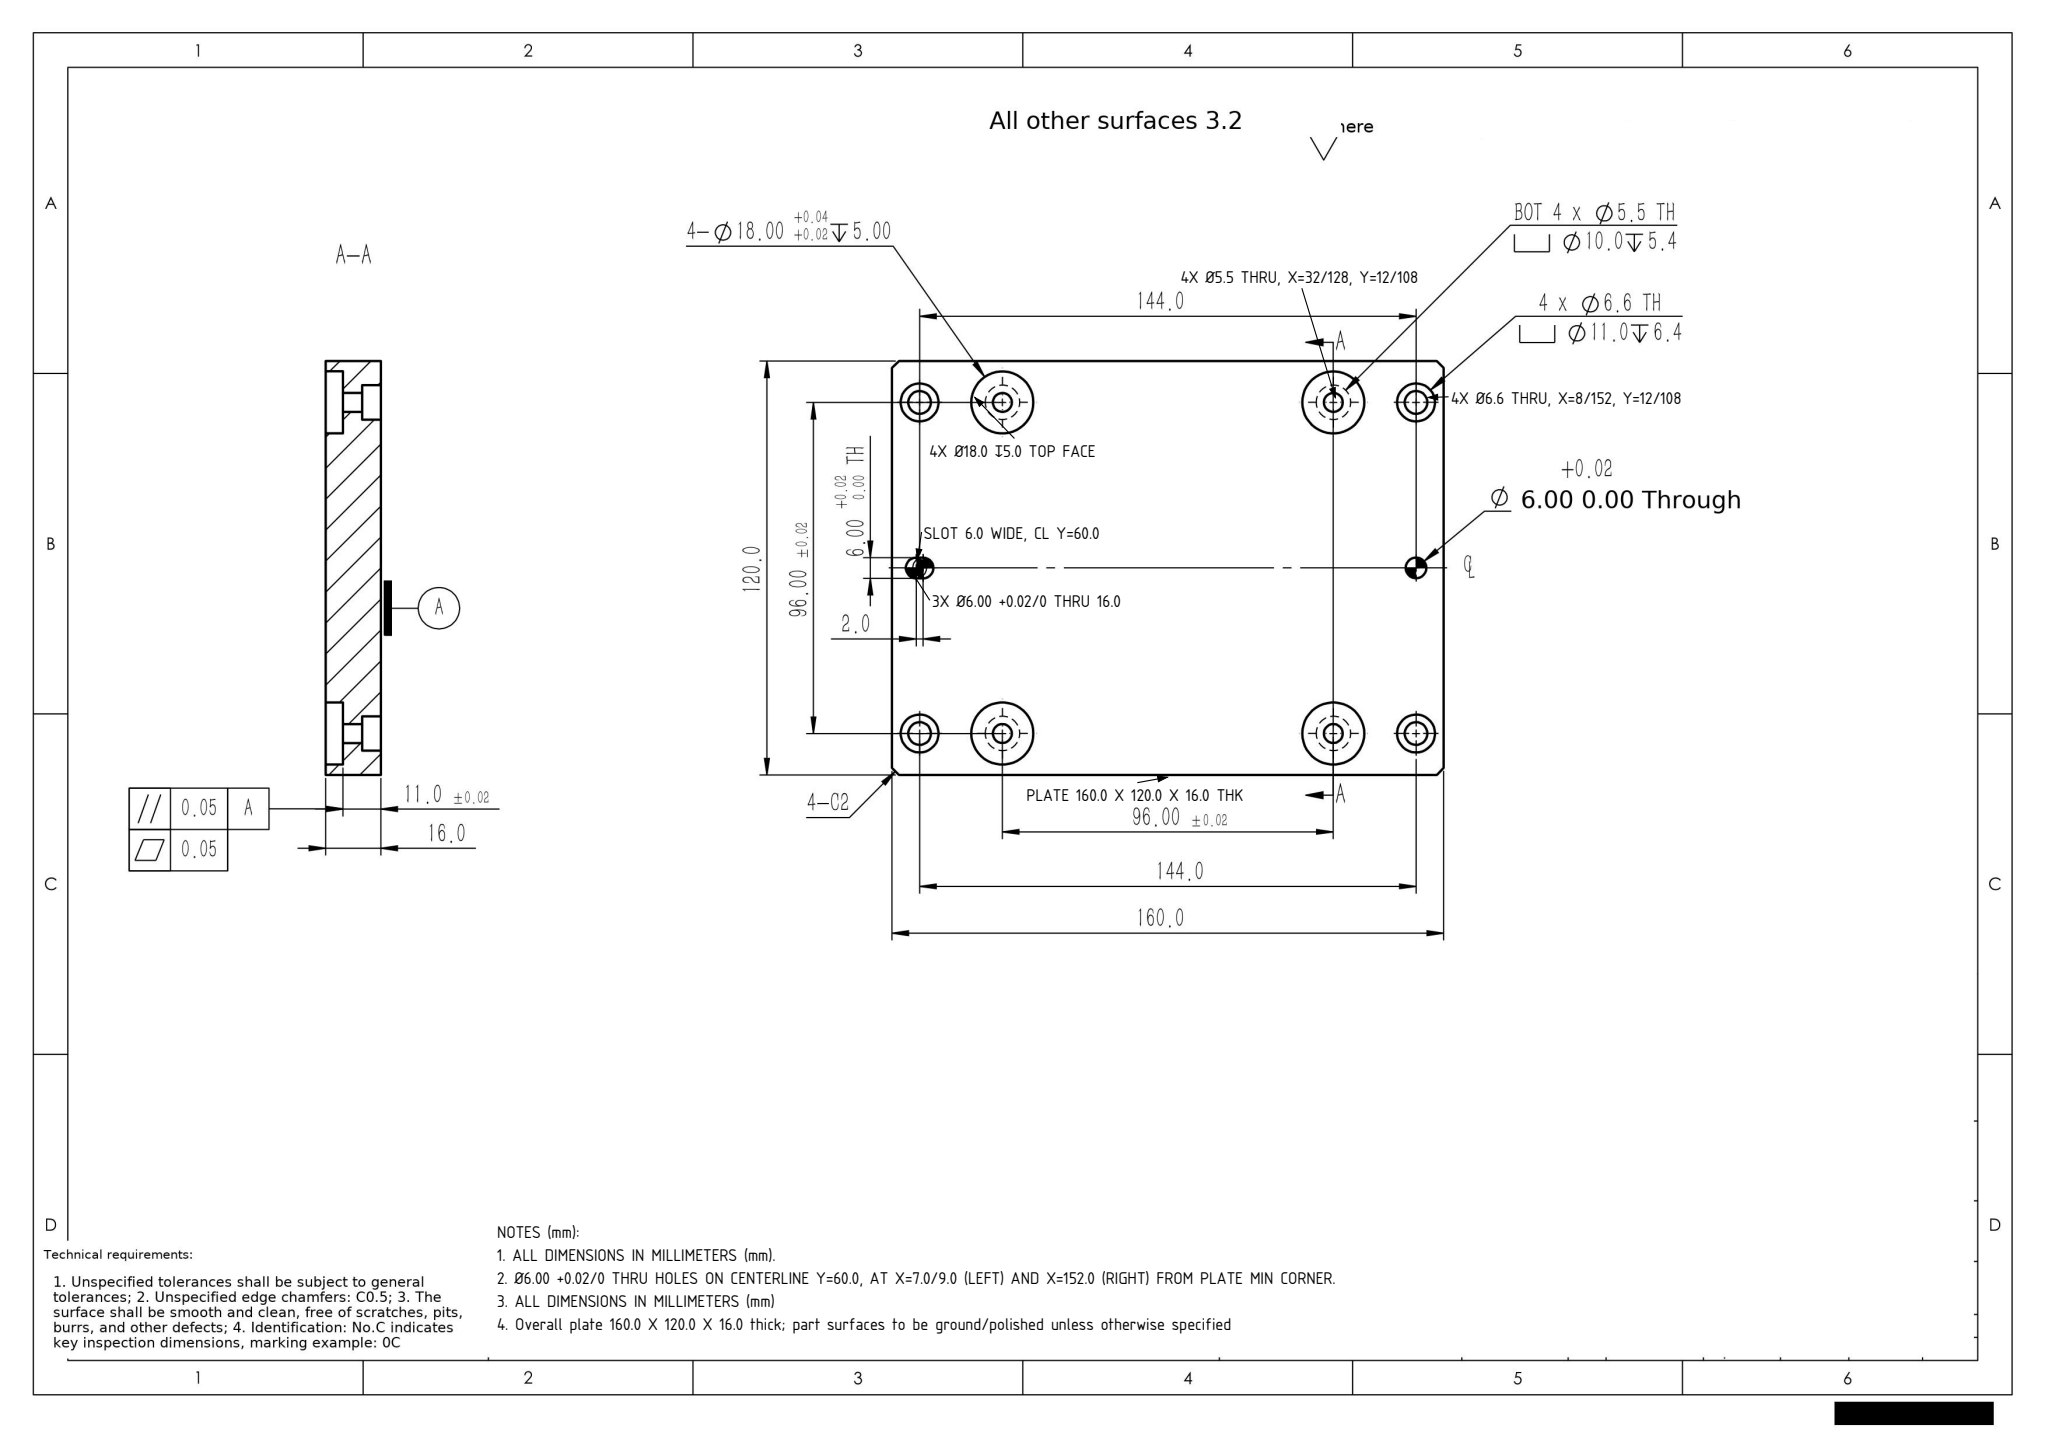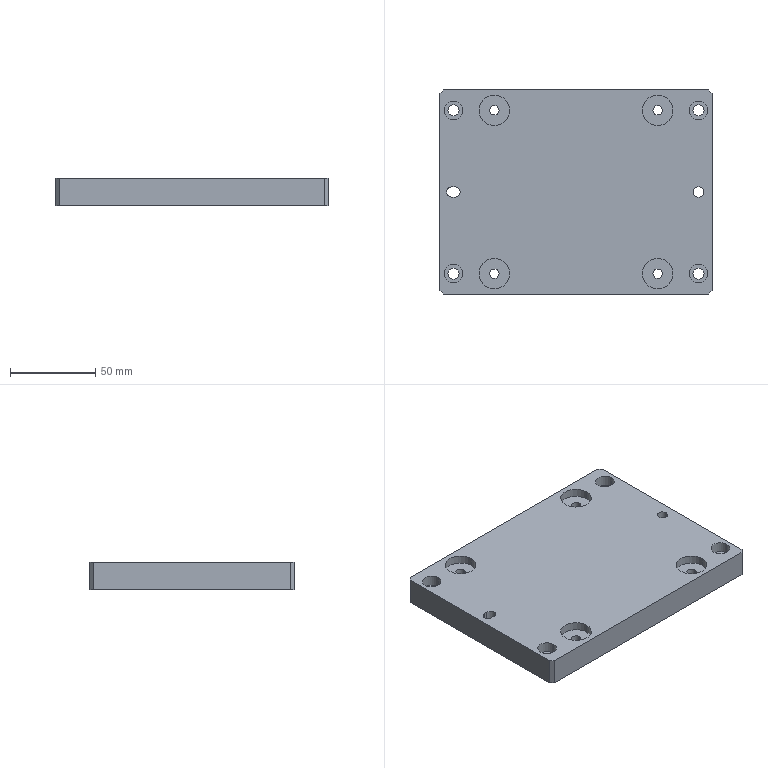Part | SolidWorks | mm | 1 solid | 69 faces | box 160 x 120 x 16 mm | volume 294911 mm3 | cylinder 45 | plane 24 | commonest cylinder face diameters 11 x8 6.6 x8 18 x8 10 x8 5.5 x8 6 x5
Drawing notes:
ALL DIMENSIONS IN MILLIMETERS (mm). | from the solid: STEP model units mm; bbox_xyz [160.0, 120.0, 16.0]
PLATE OVERALL SIZE 160.0 x 120.0 x 16.0 THICK. | from the solid: bbox_xyz [160.0, 120.0, 16.0]
4X Ø6.6 THRU, C'BORE Ø11.0 DP 6.4, FROM TOP FACE; HOLE CENTERS AT X=8.0 AND 152.0, Y=12.0 AND 108.0 FROM PLATE MIN CORNER. | from the solid: cylinders [6.6,z,(8.0/152.0, 12.0/108.0),9.6] and [11.0,z,same,6.4]
4X Ø5.5 THRU FROM BOTTOM FACE, C'BORE Ø10.0 DP 5.4; HOLE CENTERS AT X=32.0 AND 128.0, Y=12.0 AND 108.0 FROM PLATE MIN CORNER. | from the solid: cylinders [5.5,z,(32.0/128.0, 12.0/108.0),5.6] and [10.0,z,same,5.4]
4X Ø18.0 DP 5.0 COUNTERBORE IN TOP FACE, COAXIAL WITH Ø5.5 HOLES AT X=32.0 AND 128.0, Y=12.0 AND 108.0. | from the solid: cylinders [18.0,z,(32.0/128.0, 12.0/108.0),5.0]
Ø6.00 +0.02/0 THRU HOLES ON CENTERLINE Y=60.0, AT X=7.0/9.0 (LEFT) AND X=152.0 (RIGHT) FROM PLATE MIN CORNER. | from the solid: cylinders [6.0,z,(7.0,60.0),16.0], [6.0,z,(9.0,60.0),16.0], [6.0,z,(152.0,60.0),16.0]
CENTRAL SLOT/POCKET FLANKS AT Y=57.0 AND Y=63.0 (6.0 WIDE, CENTERED ON Y=60.0). | from the solid: axis_planes y=57.0 and y=63.0
ALL DIMENSIONS IN MILLIMETERS (mm) | from the solid: STEP header: units mm; bbox_xyz [160.0, 120.0, 16.0]
3X Ø6.00 +0.02/0 THRU (16.0 deep), axes parallel Z at X=7.0, X=9.0 and X=152.0, all at Y=60.0 from bbox min corner | from the solid: cylinders dia 6.0 axis z at [7.0,60.0], [9.0,60.0], [152.0,60.0], length 16.0
Overall plate 160.0 X 120.0 X 16.0 thick; part surfaces to be ground/polished unless otherwise specified | from the solid: bbox_xyz [160.0,120.0,16.0]; planes z=0.0 and z=16.0